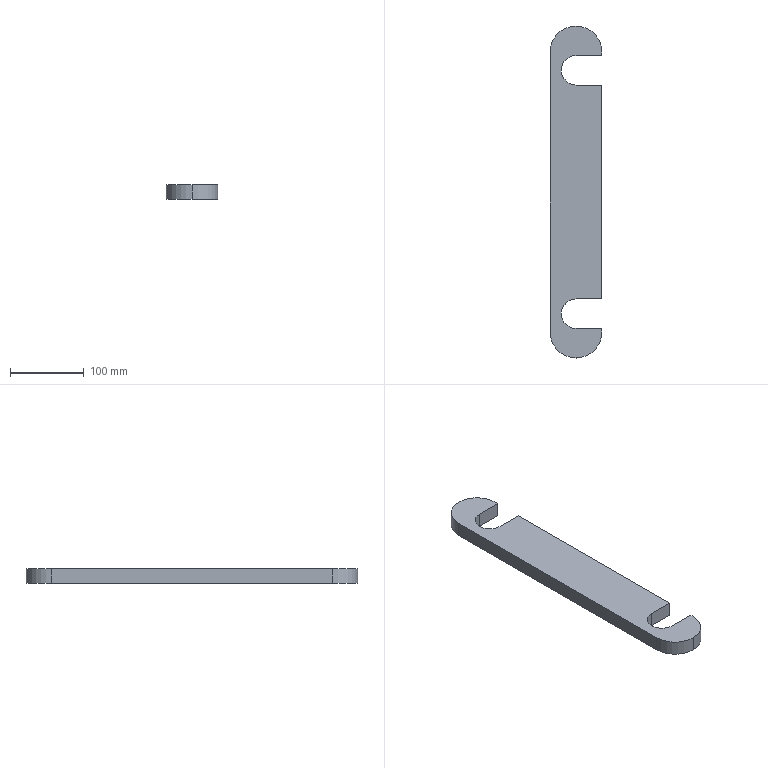Component | NX | CLAMP_PLATE_2 | 1 solid | 16 faces | volume 527836 mm3 | plane 10 | cylinder 6 | commonest cylinder face diameters 70 x4 40 x2